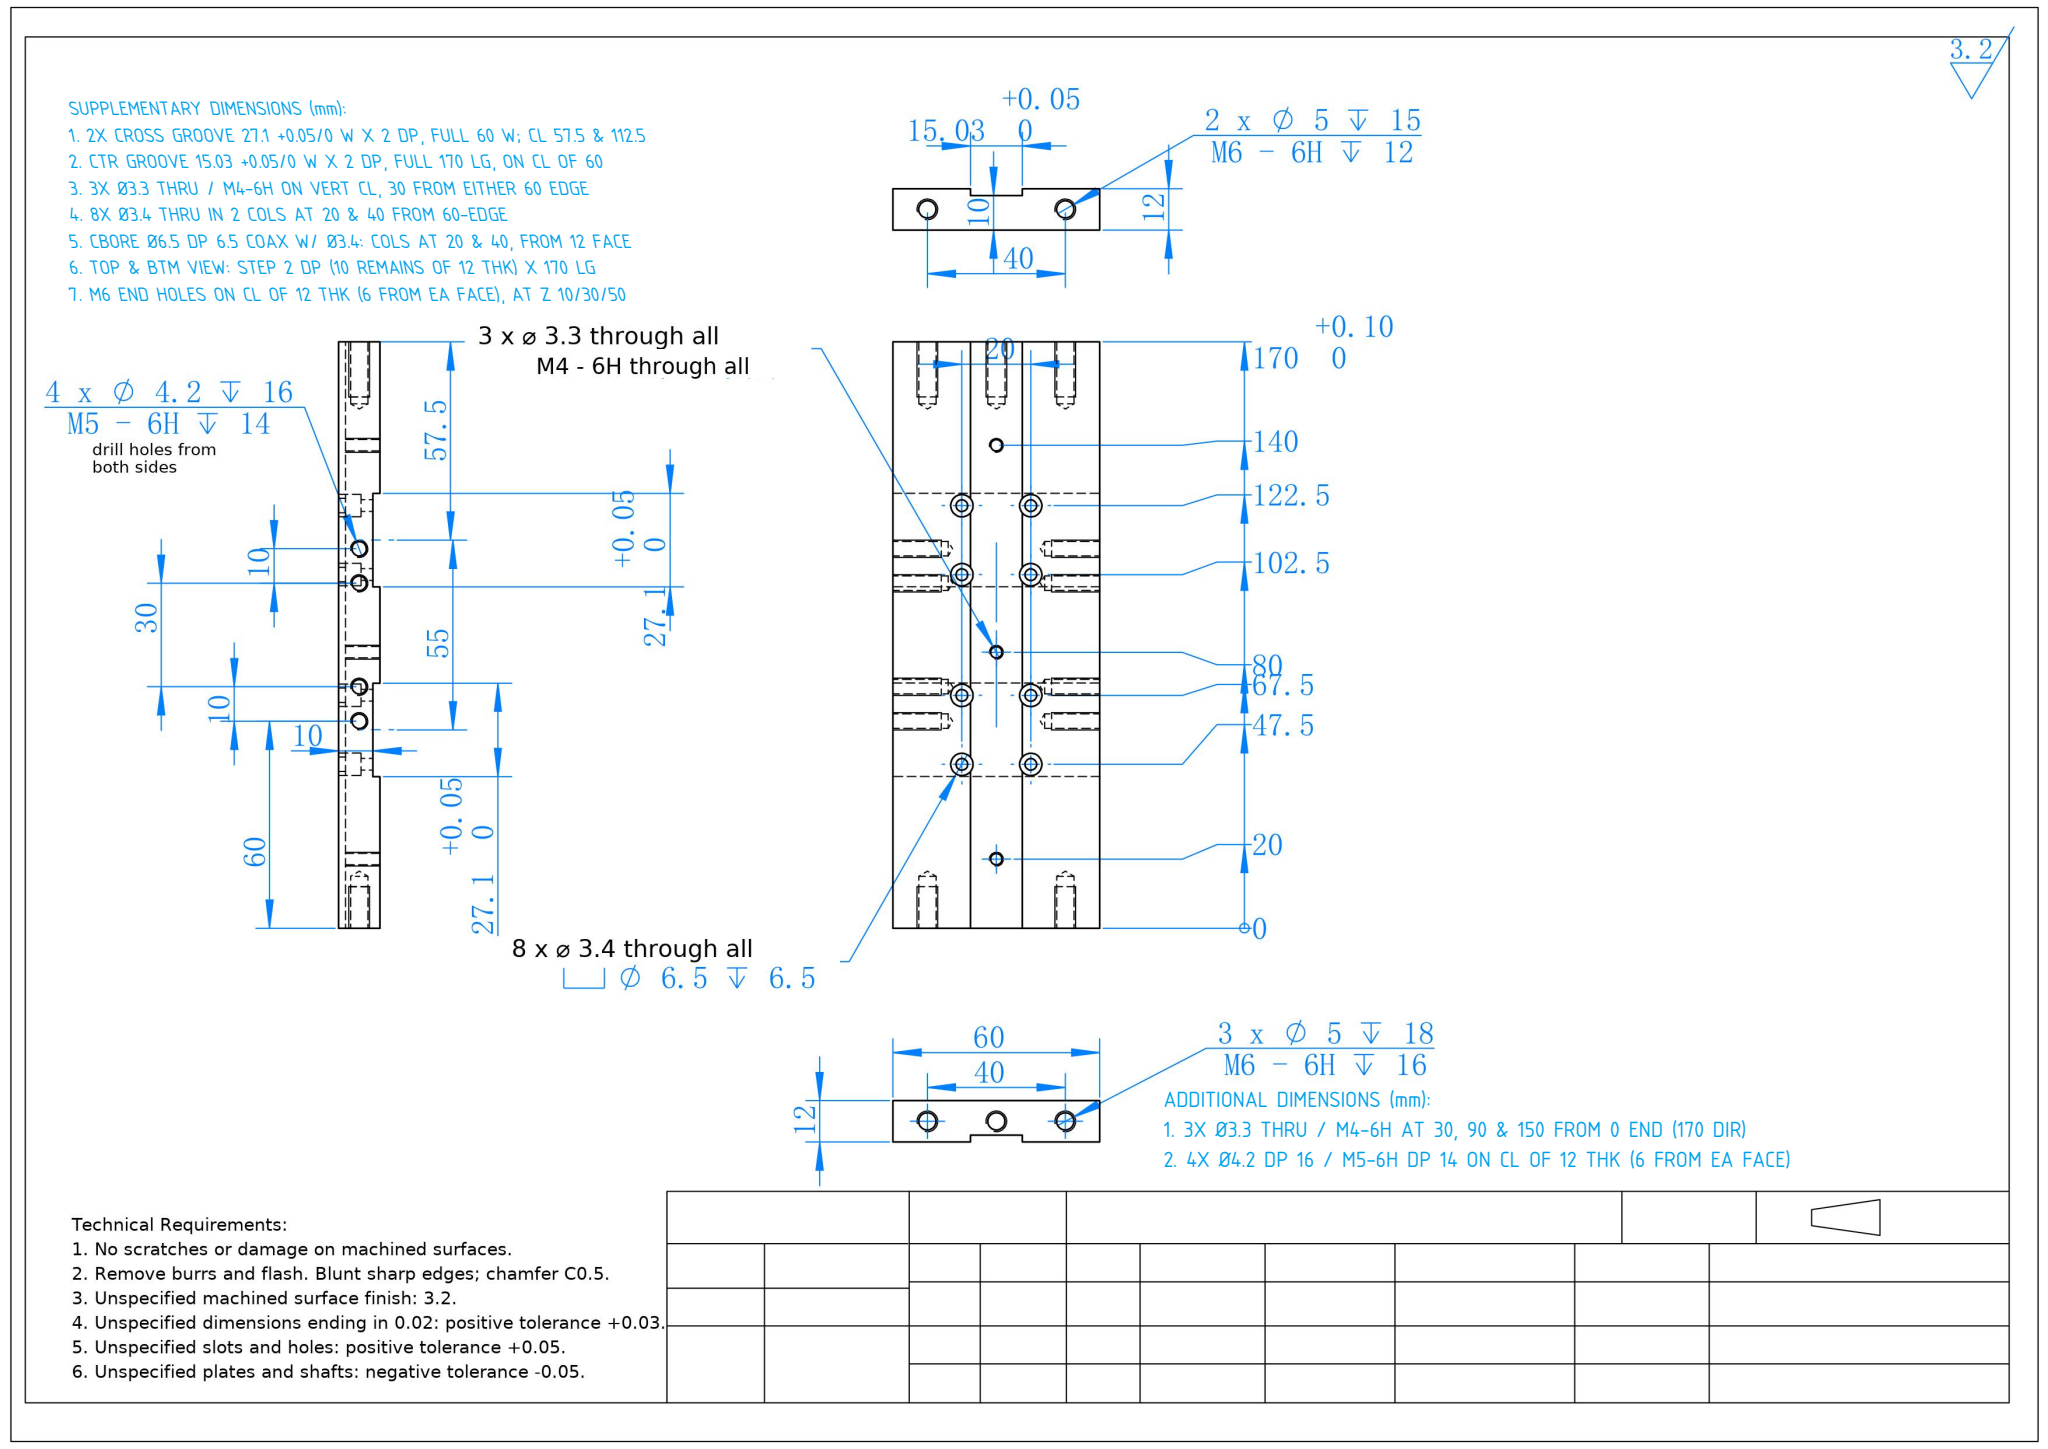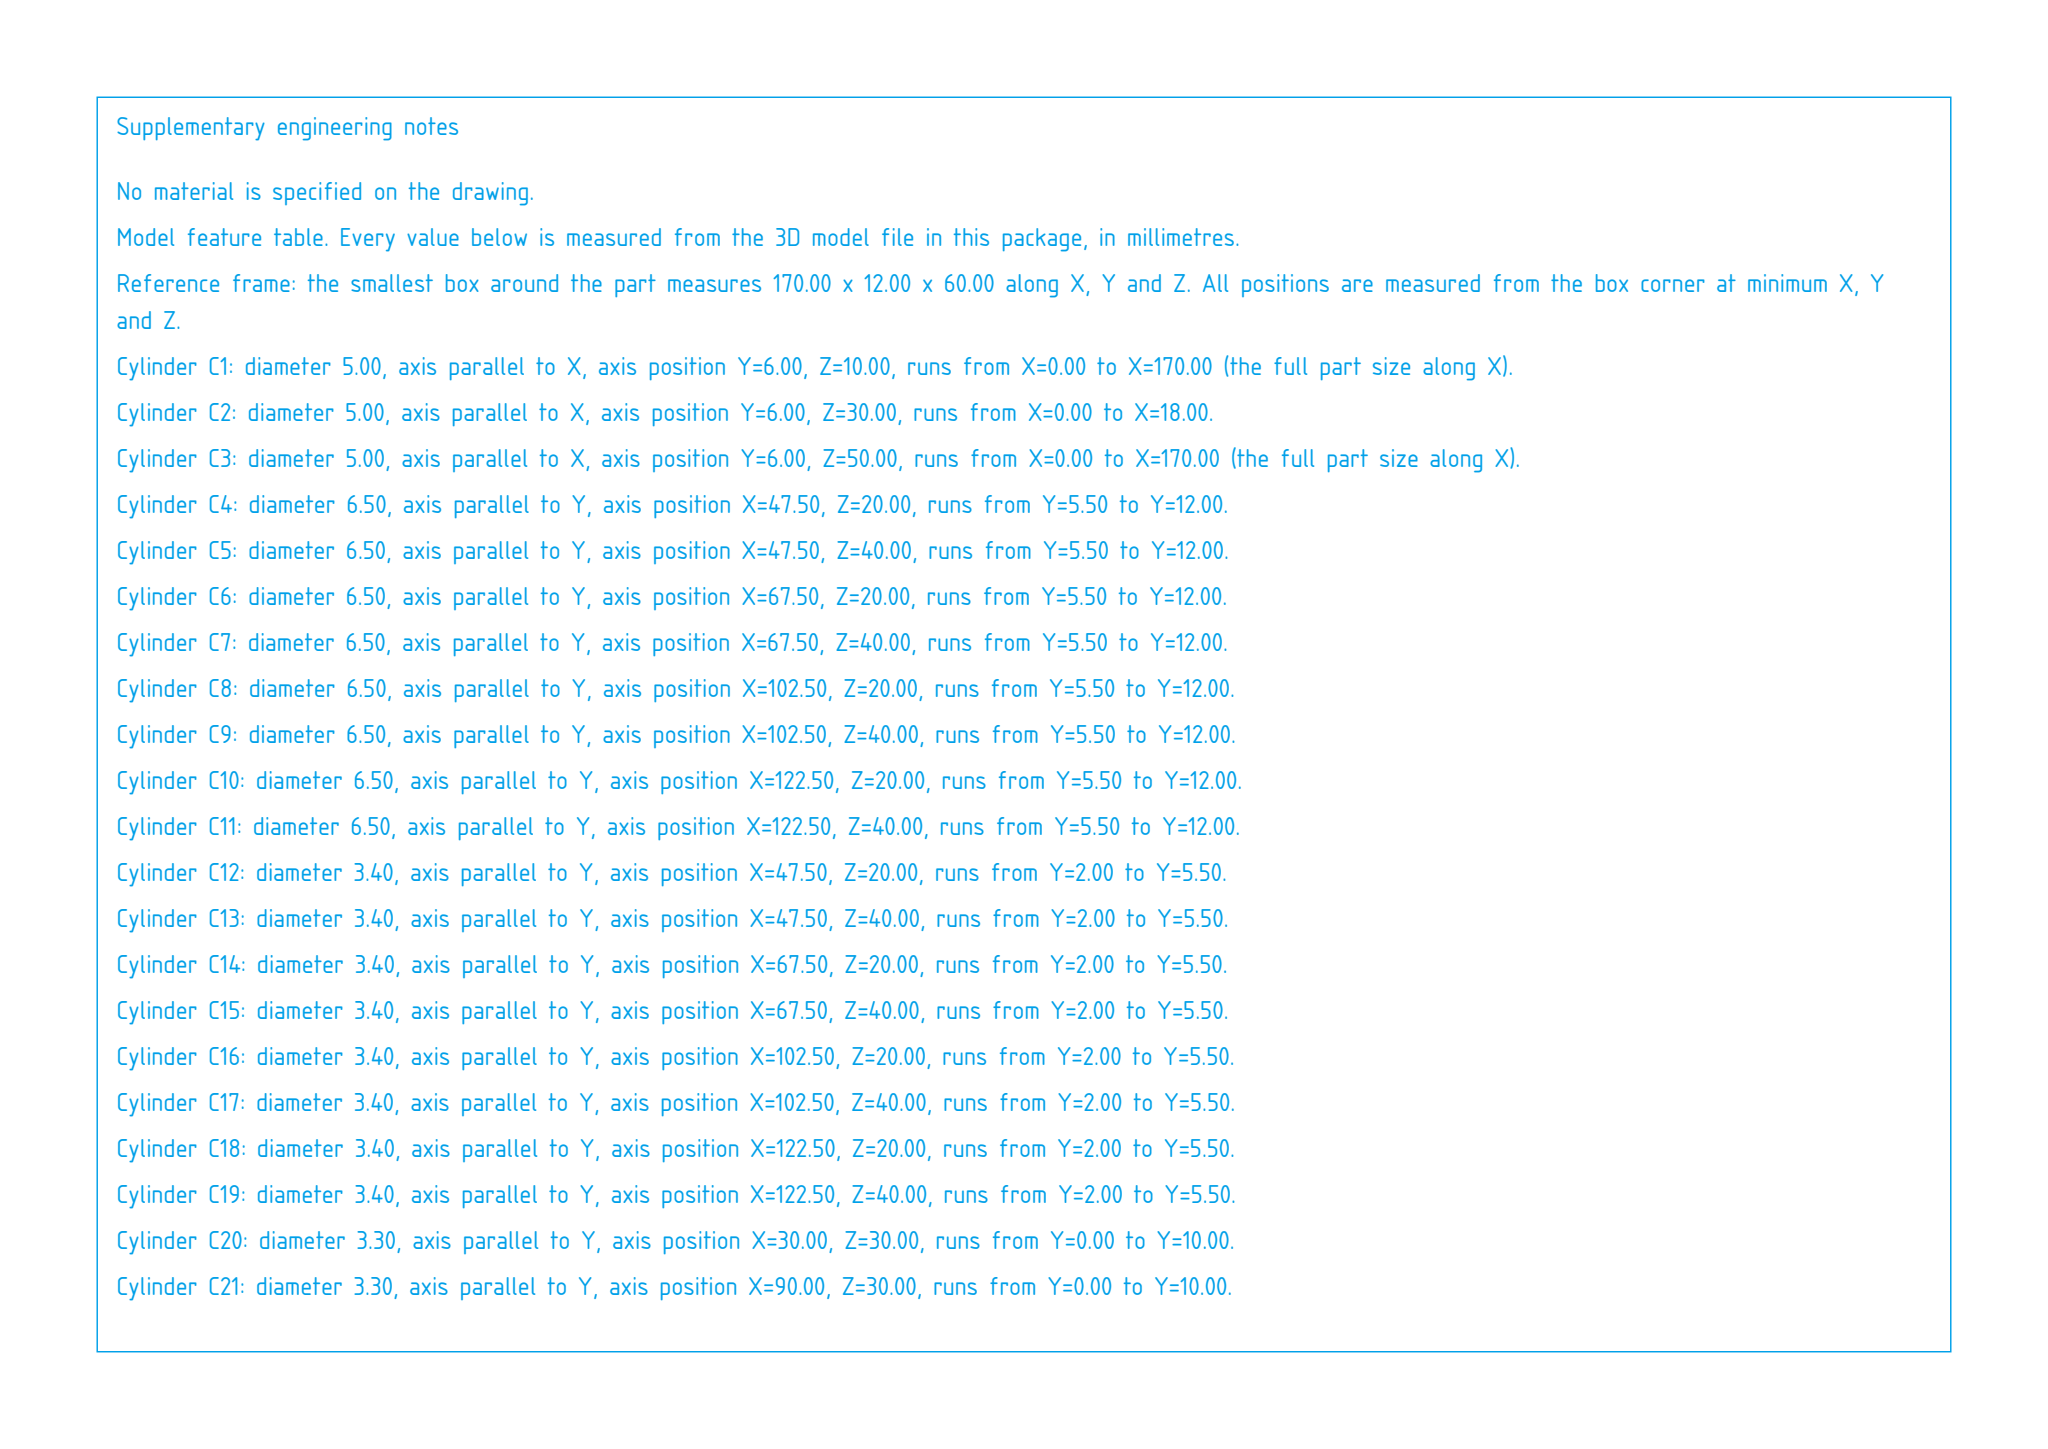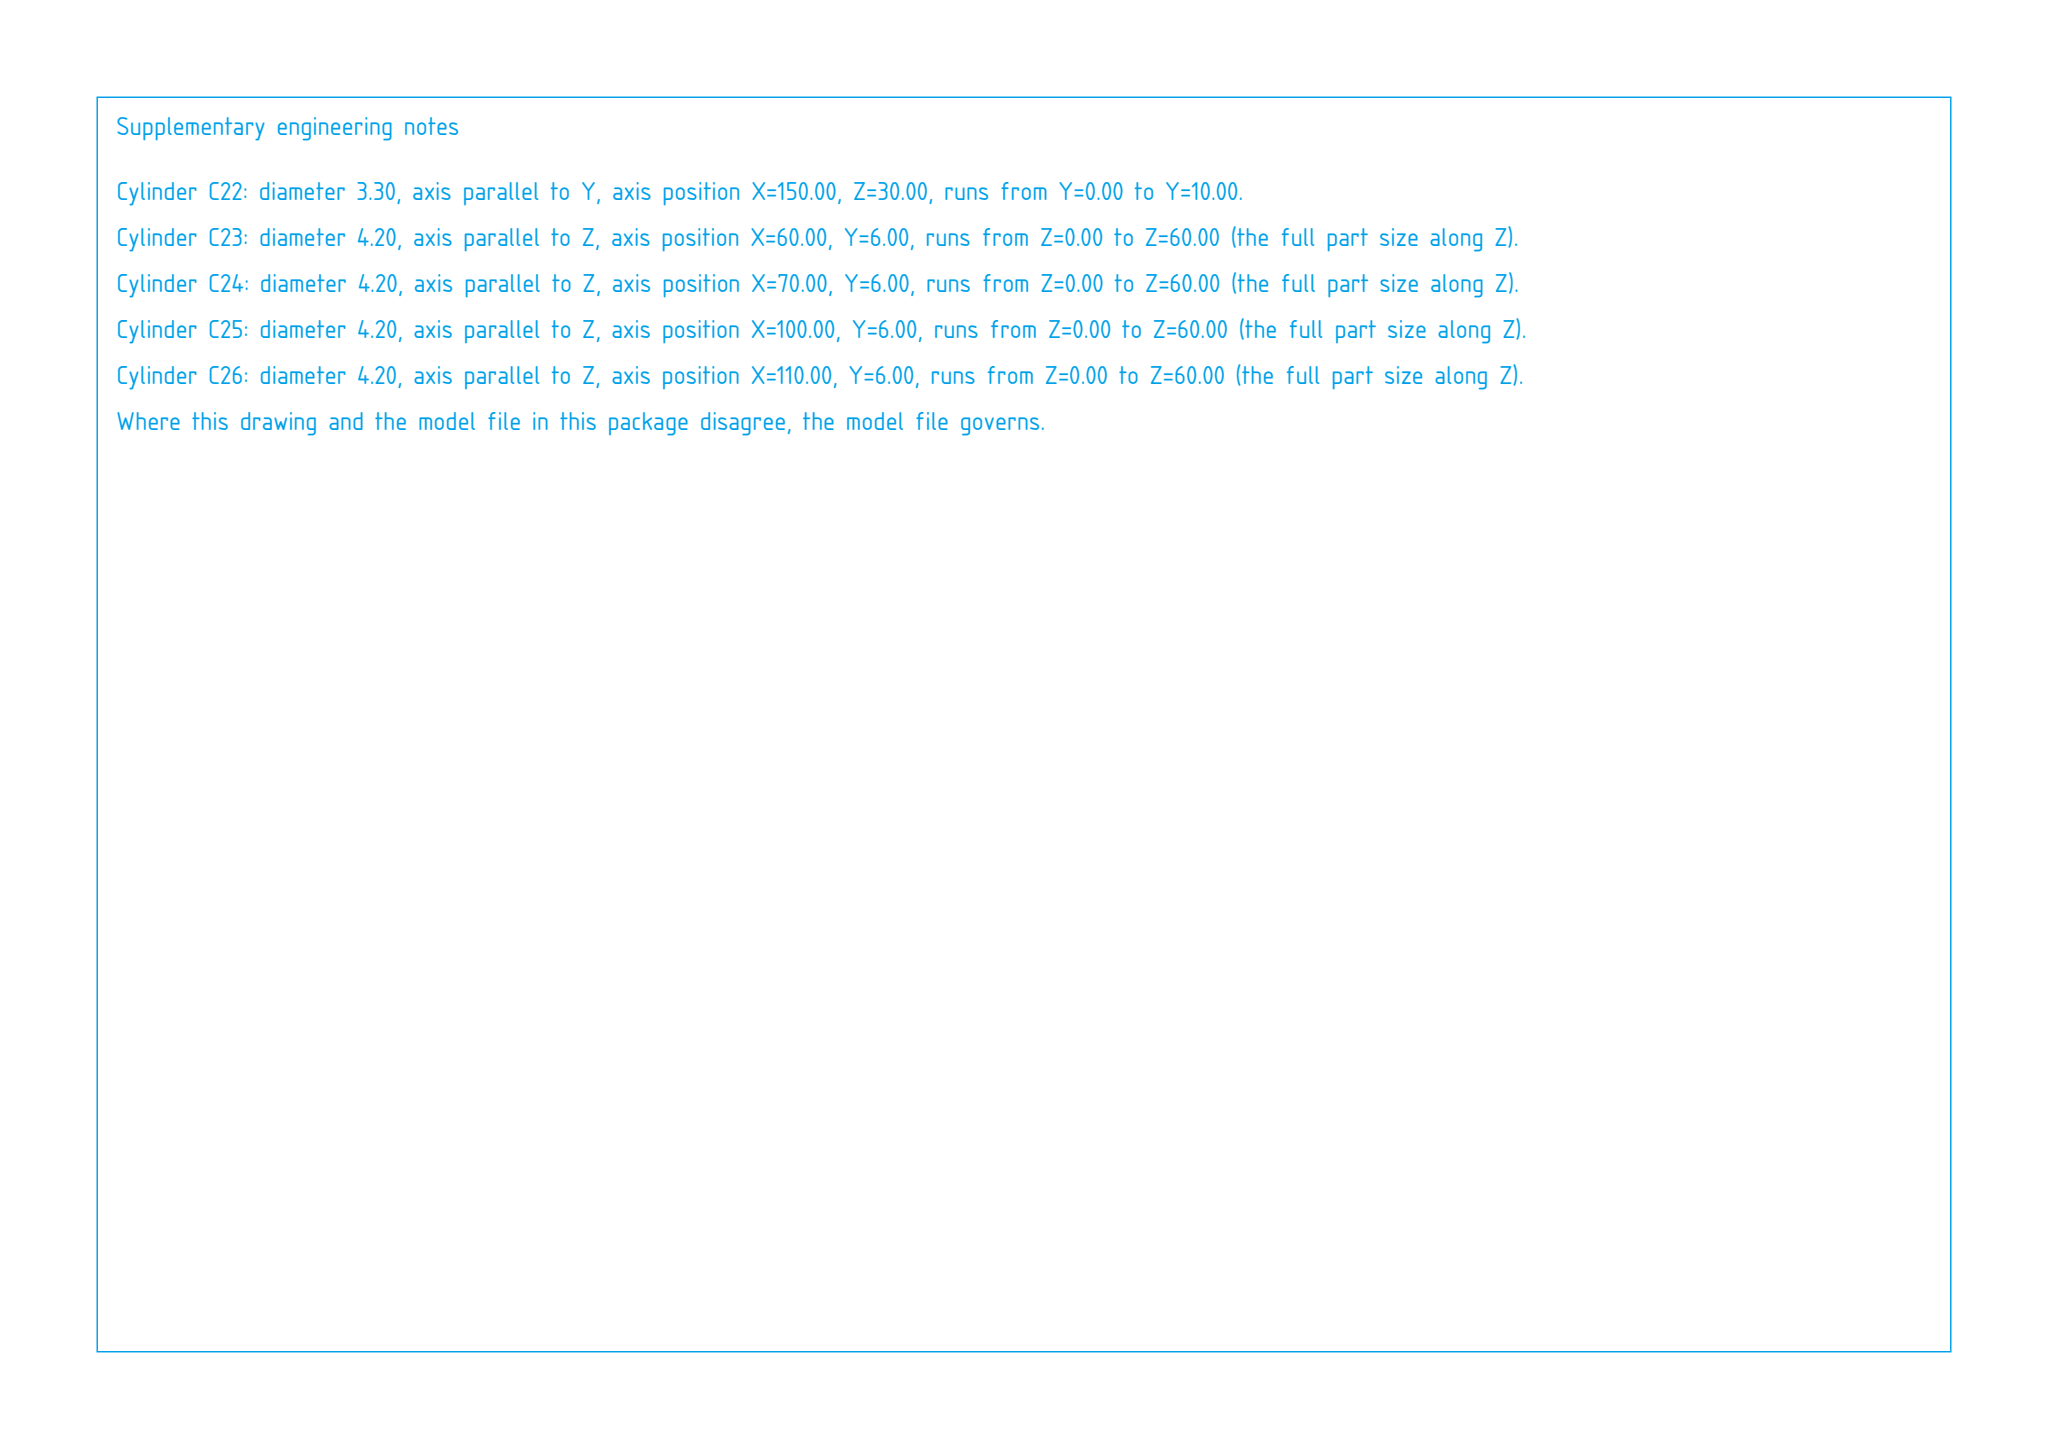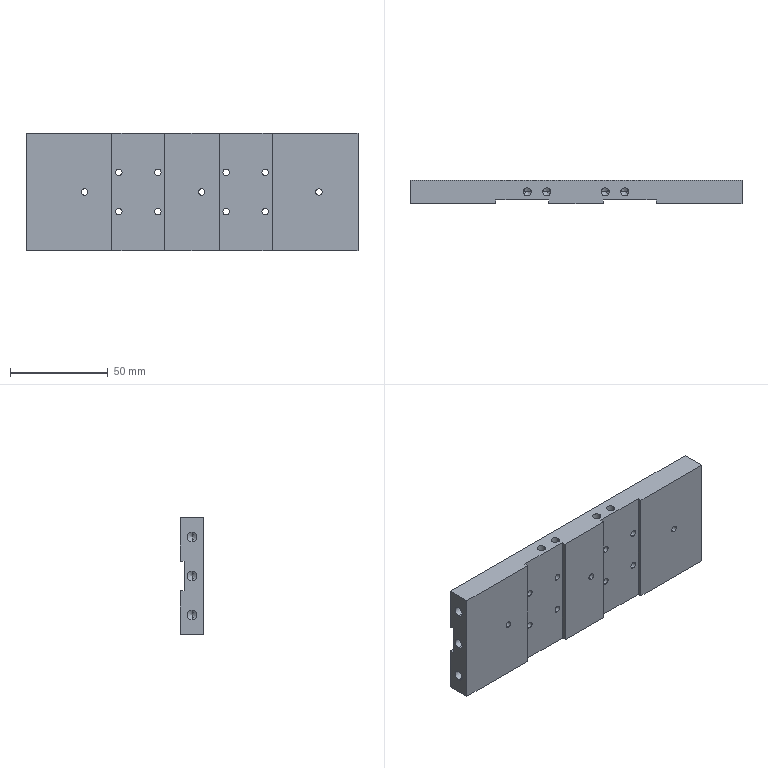Part | SolidWorks | mm | 1 solid | 124 faces | box 170 x 12 x 60 mm | volume 105066 mm3 | cylinder 64 | plane 34 | cone 26 | commonest cylinder face diameters 4.2 x16 6.5 x16 3.4 x16 5 x10 3.3 x6
build123d program:
from build123d import *

# Parameters (mm, degrees)
SKETCH1_W                                       = 170
SKETCH1_H                                       = 12
EXTRUDE1_DEPTH                                  = 30
SKETCH20_W                                      = 170
SKETCH20_H                                      = 15.03
CUT_EXTRUDE3_DEPTH                              = 2
SKETCH31_W                                      = 27.1
SKETCH31_H                                      = 60
CUT_EXTRUDE4_DEPTH                              = 2
M6_TAPPED_HOLE2_D                               = 5
M6_TAPPED_HOLE2_DEPTH                           = 18
M6_TAPPED_HOLE2_TIP                             = 1.502
M4_TAPPED_HOLE1_D                               = 3.3
M3_HEX_SOCKET_HEAD_CAP_SCREW_CBORE1_D           = 3.4
M3_HEX_SOCKET_HEAD_CAP_SCREW_CBORE1_CBORE_D     = 6.5
M3_HEX_SOCKET_HEAD_CAP_SCREW_CBORE1_CBORE_DEPTH = 6.5
M6_TAPPED_HOLE1_D                               = 5
M6_TAPPED_HOLE1_DEPTH                           = 15
M6_TAPPED_HOLE1_TIP                             = 1.502
M5_TAPPED_HOLE1_D                               = 4.2
M5_TAPPED_HOLE1_DEPTH                           = 16
M5_TAPPED_HOLE1_TIP                             = 1.262
M5_TAPPED_HOLE3_D                               = 4.2
M5_TAPPED_HOLE3_DEPTH                           = 16
M5_TAPPED_HOLE3_TIP                             = 1.262


with BuildPart() as part:
    # Sketch1 → Extrude1 (new, symmetric)
    with BuildSketch(Plane.XY):
        Rectangle(SKETCH1_W, SKETCH1_H)
    extrude(amount=EXTRUDE1_DEPTH, both=True)

    # Sketch20 → Cut-Extrude3 (cut)
    with BuildSketch(Plane(origin=(0, 6, 0), x_dir=(-1, 0, 0), z_dir=(0, 1, 0))):
        Rectangle(SKETCH20_W, SKETCH20_H)
    extrude(amount=-CUT_EXTRUDE3_DEPTH, mode=Mode.SUBTRACT)

    # Sketch31 → Cut-Extrude4 (cut)
    with BuildSketch(Plane(origin=(0, -6, 0), x_dir=(-1, 0, 0), z_dir=(0, -1, 0))):
        with Locations((27.5, 0)):
            Rectangle(SKETCH31_W, SKETCH31_H)
        with Locations((-27.5, 0)):
            Rectangle(SKETCH31_W, SKETCH31_H)
    extrude(amount=-CUT_EXTRUDE4_DEPTH, mode=Mode.SUBTRACT)

    # M6 Tapped Hole2
    with Locations(Plane.ZY.offset(85)):
        with Locations((-20, 0), (20, 0), (0, 0)):
            Hole(M6_TAPPED_HOLE2_D / 2, depth=M6_TAPPED_HOLE2_DEPTH)
            with Locations((0, 0, -(M6_TAPPED_HOLE2_DEPTH + M6_TAPPED_HOLE2_TIP / 2))):  # 118° drill point
                Cone(0, M6_TAPPED_HOLE2_D / 2, M6_TAPPED_HOLE2_TIP, mode=Mode.SUBTRACT)

    # M4 Tapped Hole1 (through all)
    with Locations(Plane(origin=(0, 6, 0), x_dir=(1, 0, 0), z_dir=(0, 1, 0))):
        with Locations((5, 0), (65, 0), (-55, 0)):
            Hole(M4_TAPPED_HOLE1_D / 2)

    # M3 Hex Socket Head Cap Screw CBORE1 (through all)
    with Locations(Plane(origin=(0, 6, 0), x_dir=(1, 0, 0), z_dir=(0, 1, 0))):
        with Locations((-37.5, 10), (-17.5, 10), (-37.5, -10), (-17.5, -10), (17.5, 10), (37.5, 10), (17.5, -10), (37.5, -10)):
            CounterBoreHole(M3_HEX_SOCKET_HEAD_CAP_SCREW_CBORE1_D / 2, M3_HEX_SOCKET_HEAD_CAP_SCREW_CBORE1_CBORE_D / 2, M3_HEX_SOCKET_HEAD_CAP_SCREW_CBORE1_CBORE_DEPTH)

    # M6 Tapped Hole1
    with Locations(Plane(origin=(85, 0, 0), x_dir=(0, 0, -1), z_dir=(1, 0, 0))):
        with Locations((-20, 0), (20, 0)):
            Hole(M6_TAPPED_HOLE1_D / 2, depth=M6_TAPPED_HOLE1_DEPTH)
            with Locations((0, 0, -(M6_TAPPED_HOLE1_DEPTH + M6_TAPPED_HOLE1_TIP / 2))):  # 118° drill point
                Cone(0, M6_TAPPED_HOLE1_D / 2, M6_TAPPED_HOLE1_TIP, mode=Mode.SUBTRACT)

    # M5 Tapped Hole1
    with Locations(Plane(origin=(0, 0, -30), x_dir=(1, 0, 0), z_dir=(0, 0, -1))):
        with Locations((-15, 0), (15, 0), (25, 0), (-25, 0)):
            Hole(M5_TAPPED_HOLE1_D / 2, depth=M5_TAPPED_HOLE1_DEPTH)
            with Locations((0, 0, -(M5_TAPPED_HOLE1_DEPTH + M5_TAPPED_HOLE1_TIP / 2))):  # 118° drill point
                Cone(0, M5_TAPPED_HOLE1_D / 2, M5_TAPPED_HOLE1_TIP, mode=Mode.SUBTRACT)

    # M5 Tapped Hole3
    with Locations(Plane.XY.offset(30)):
        with Locations((15, 0), (-15, 0), (-25, 0), (25, 0)):
            Hole(M5_TAPPED_HOLE3_D / 2, depth=M5_TAPPED_HOLE3_DEPTH)
            with Locations((0, 0, -(M5_TAPPED_HOLE3_DEPTH + M5_TAPPED_HOLE3_TIP / 2))):  # 118° drill point
                Cone(0, M5_TAPPED_HOLE3_D / 2, M5_TAPPED_HOLE3_TIP, mode=Mode.SUBTRACT)


solid = part.part